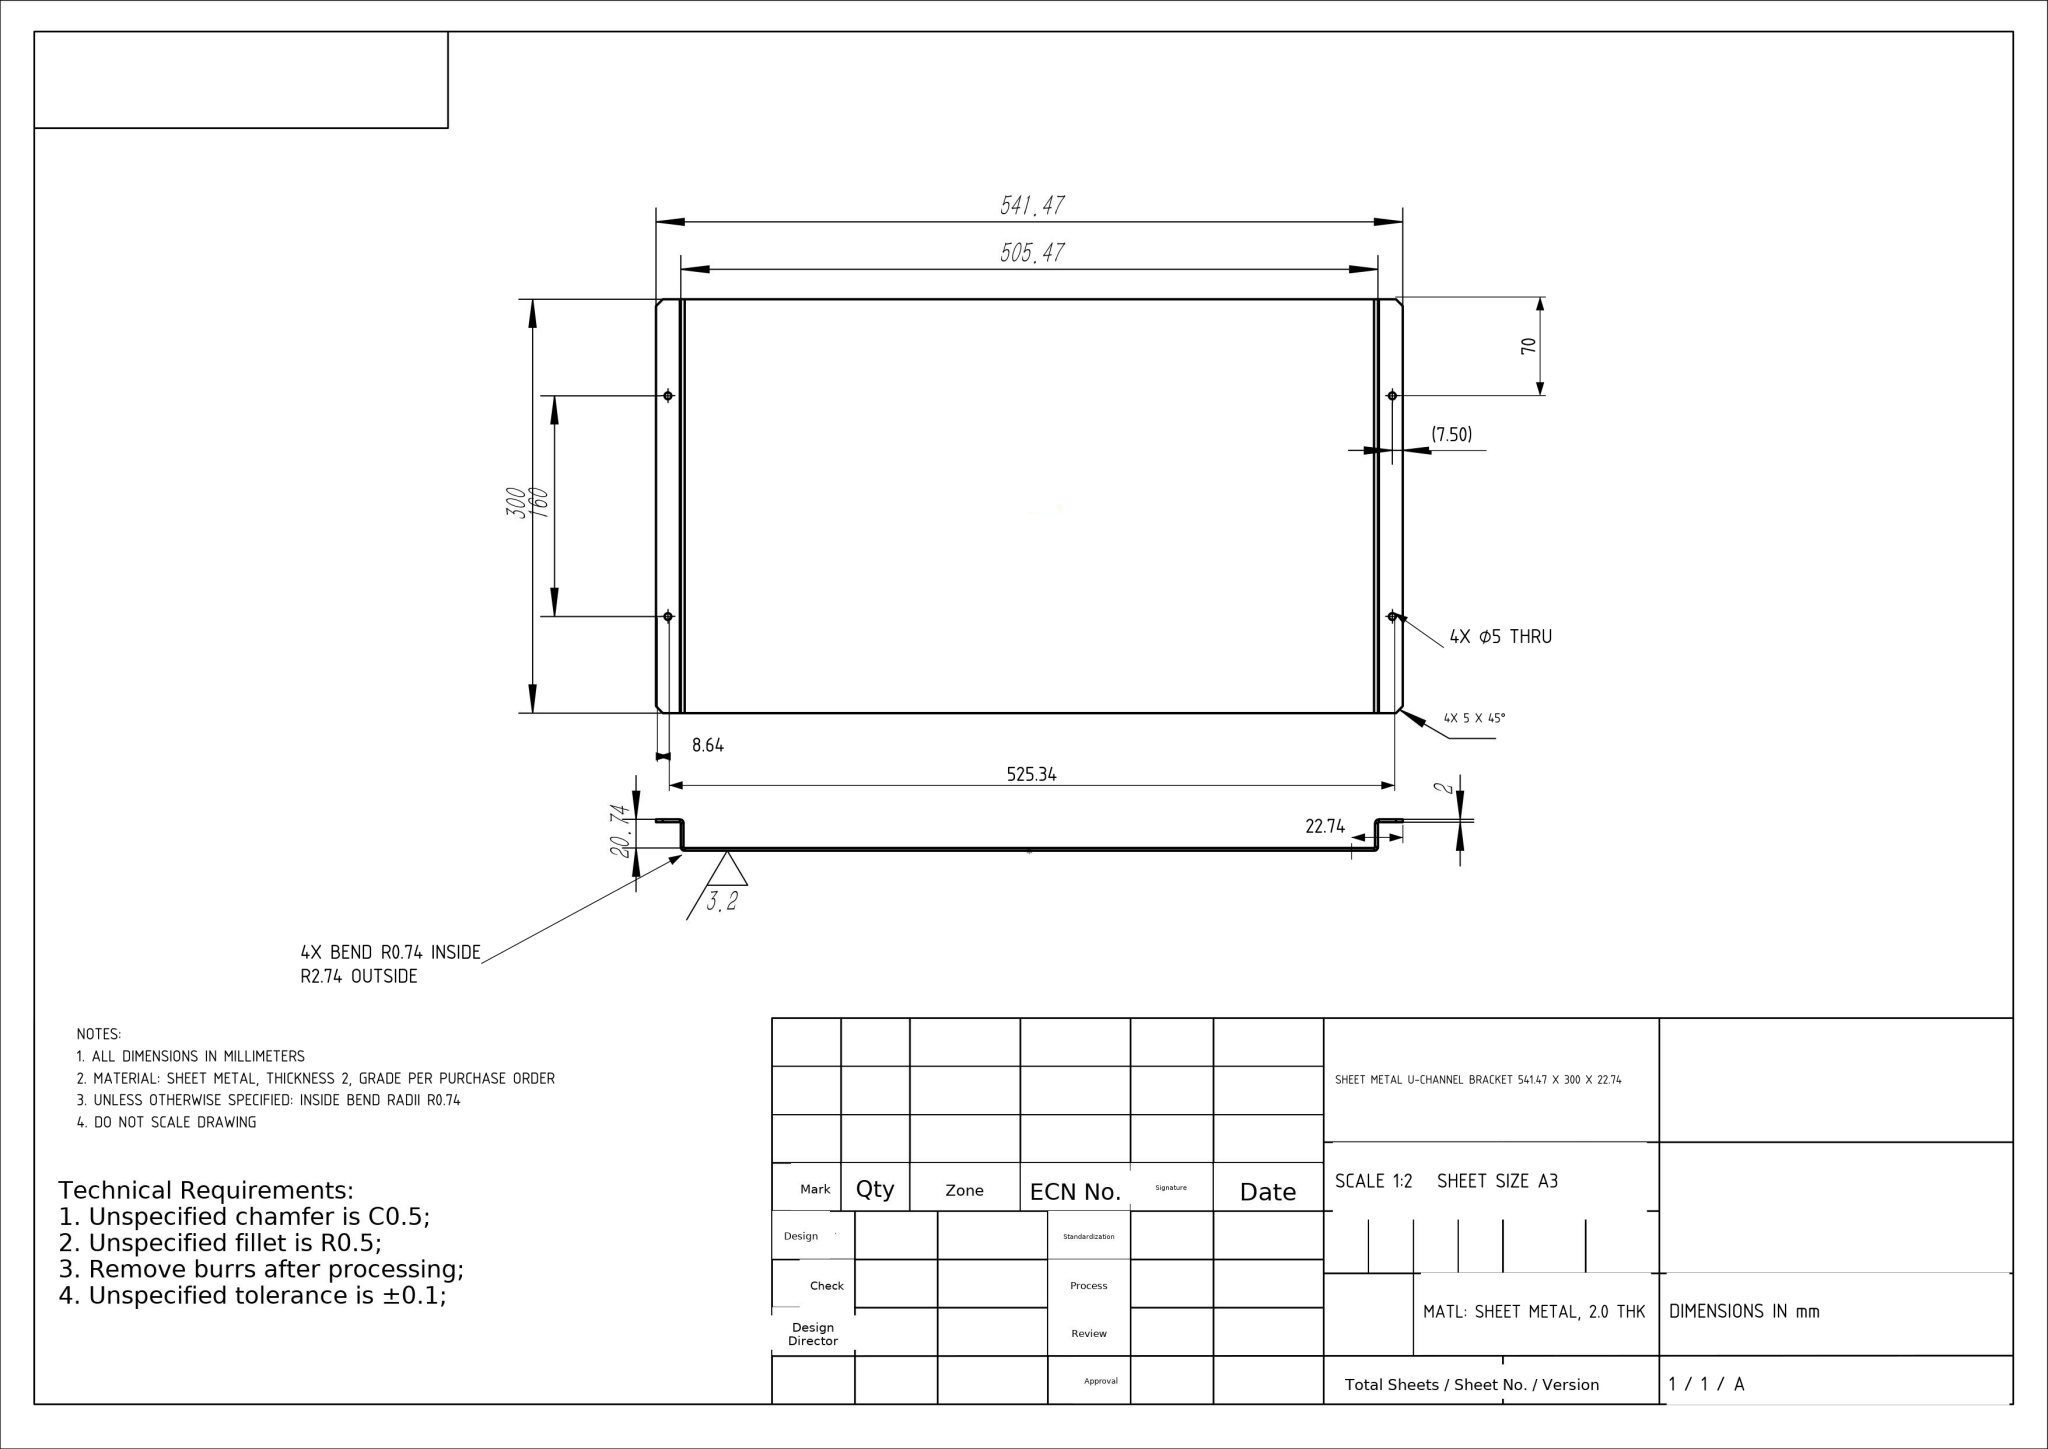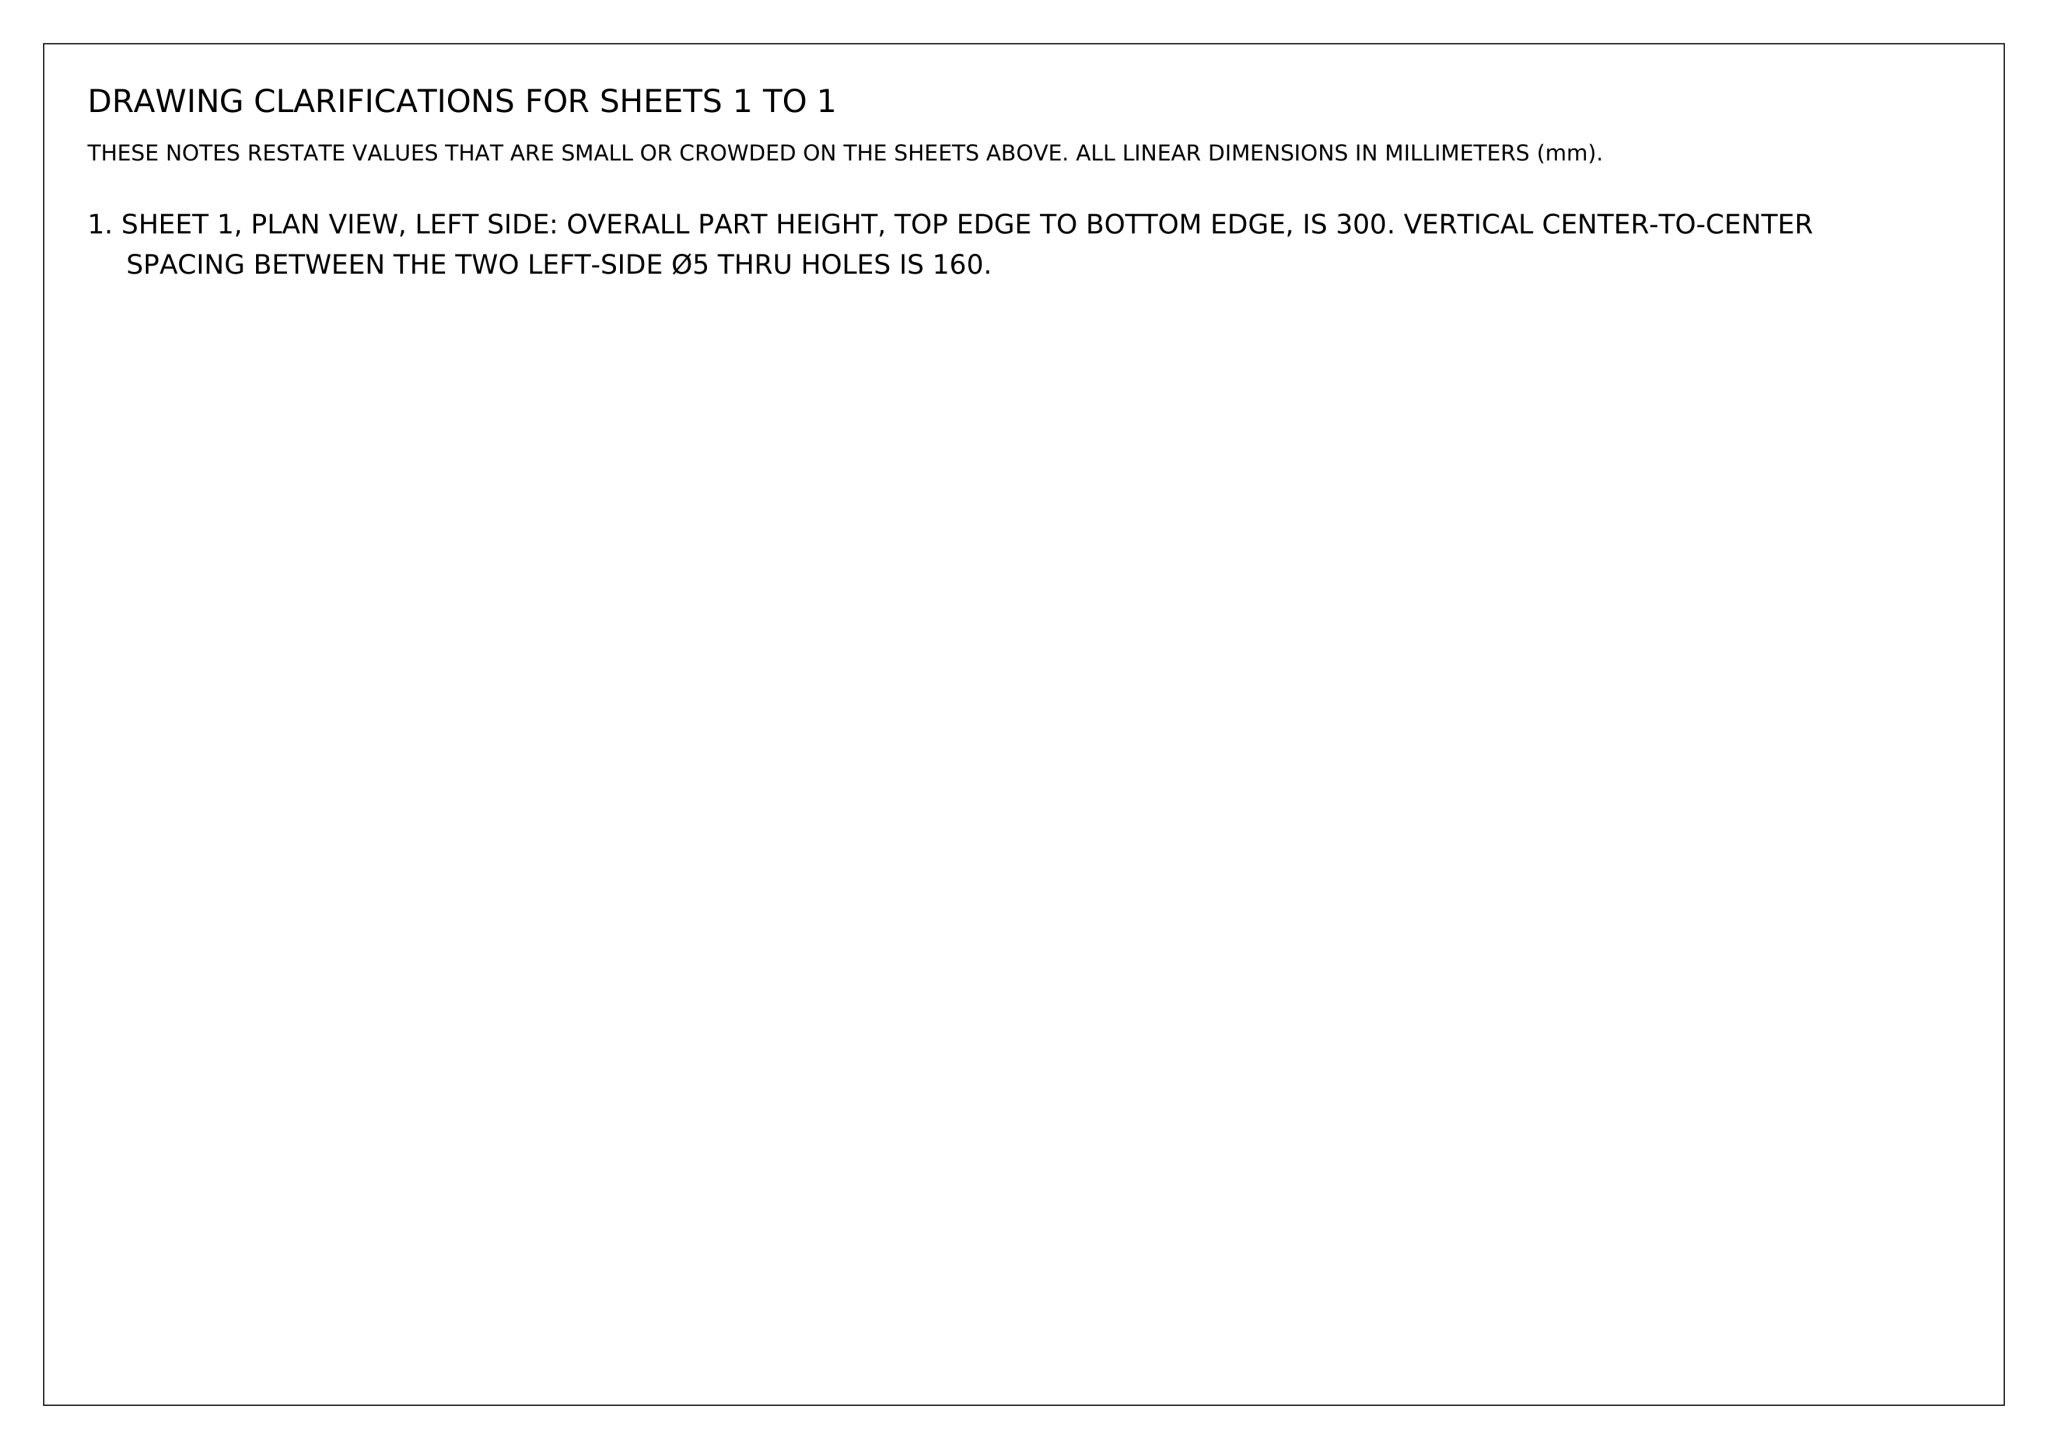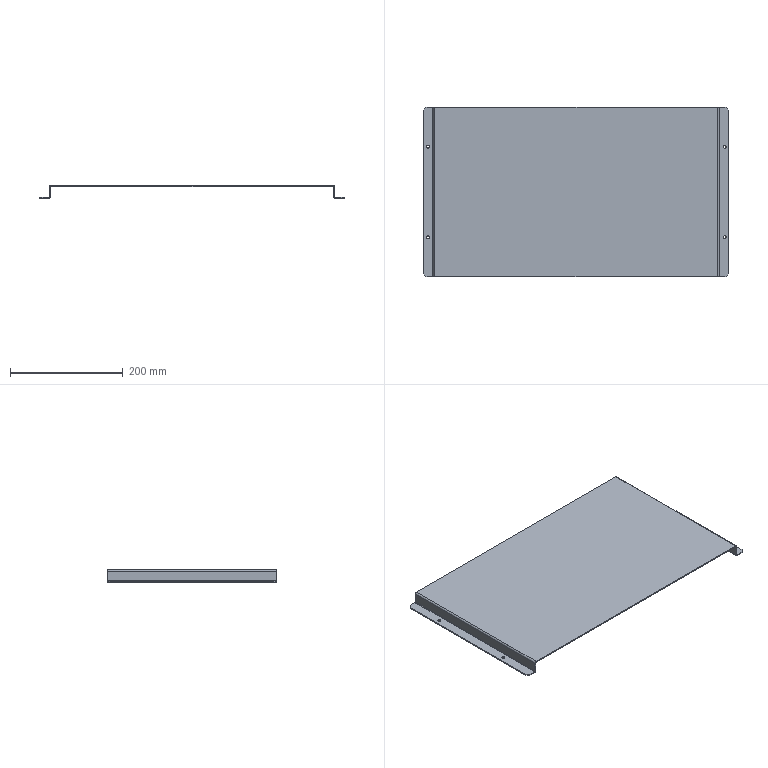Part | NX | mm | 1 solid | 50 faces | box 541.47 x 300 x 22.74 mm | volume 347722 mm3 | plane 34 | cylinder 16 | commonest cylinder face diameters 5 x8 5.473 x4 1.473 x4